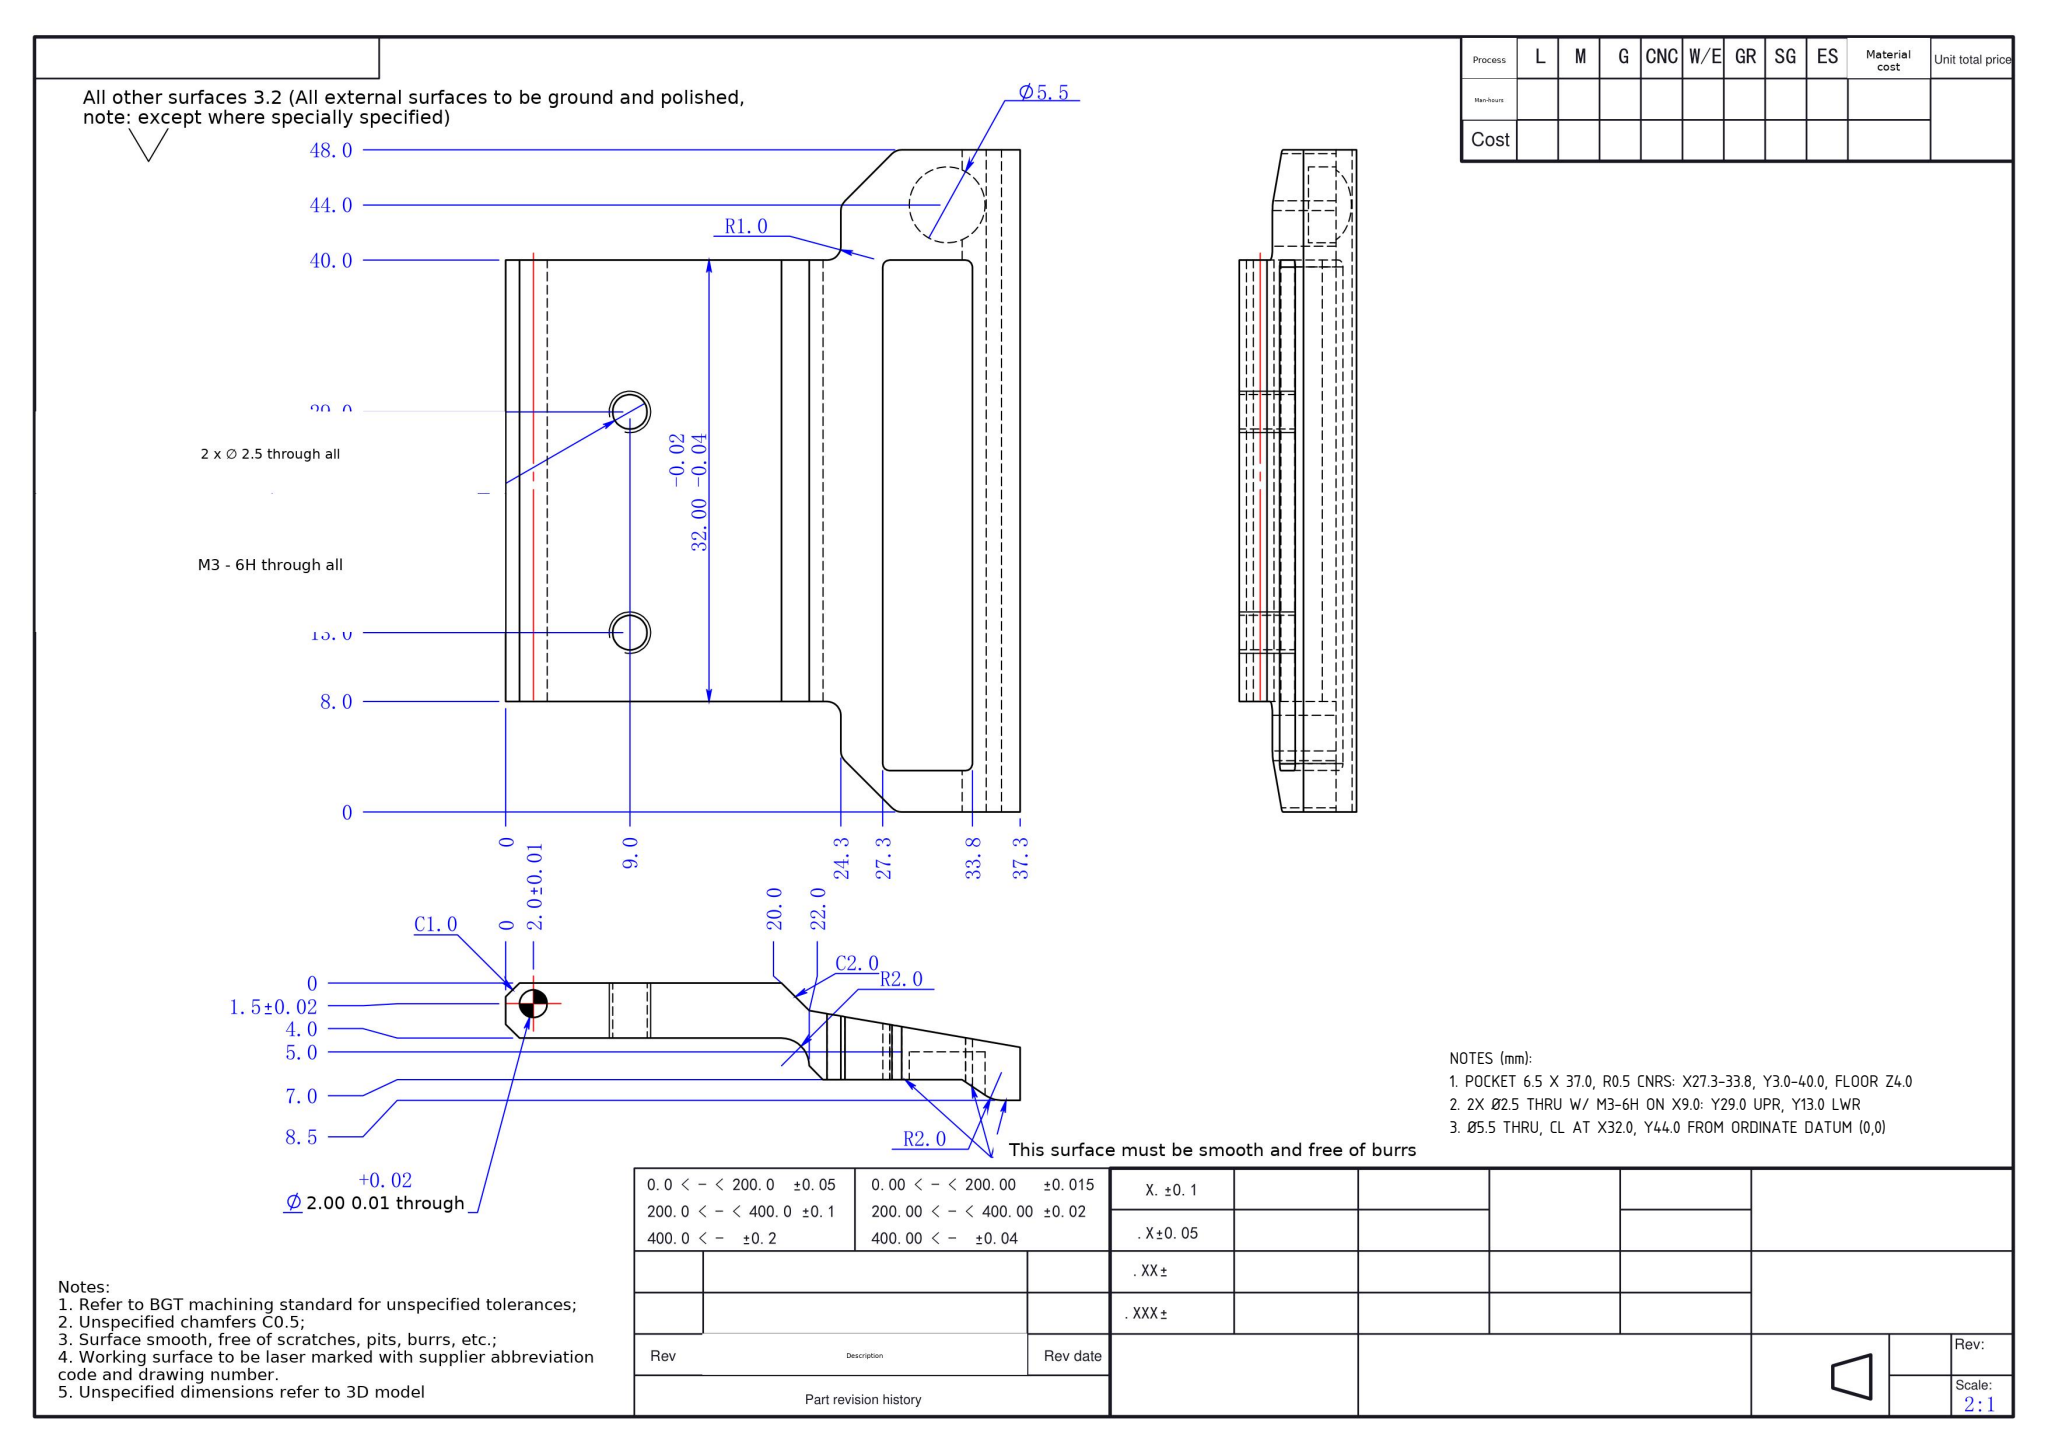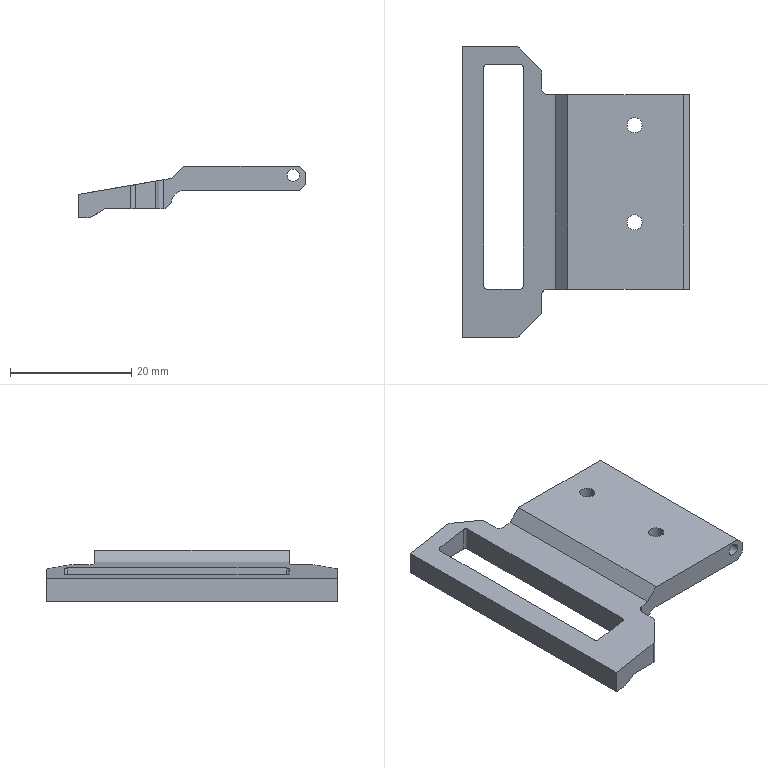Part | SolidWorks | mm | 1 solid | 45 faces | box 37.3 x 48 x 8.5 mm | volume 4364 mm3 | plane 25 | cylinder 20 | commonest cylinder face diameters 2 x8 2.5 x4 1 x4 5.5 x2 4 x2
Drawing notes:
POCKET 6.5 X 37.0, R0.5 CNRS: X27.3-33.8, Y3.0-40.0, FLOOR Z4.0 | from the solid: Ø1.0 (R0.5) cnr cyls at (3.96,8.5),(3.96,44.5),(9.46,8.5),(9.46,44.5); x-planes 3.46/9.96 -> X33.8/27.3; y-planes 8.0/45.0 -> Y40.0/3.0; z-plane 4.5 -> floor Z4.0
2X Ø2.5 THRU W/ M3-6H ON X9.0: Y29.0 UPR, Y13.0 LWR | from the solid: Ø2.5 THRU cyls, axis Z at (28.3,19.0) & (28.3,35.0); X=37.3-28.3=9.0, Y=48-19=29.0, Y=48-35=13.0
Ø5.5 THRU, CL AT X32.0, Y44.0 FROM ORDINATE DATUM (0,0) | from the solid: Ø5.5 cyl, axis Z at bbox (5.3,4.0); drawing datum flip: X=37.3-5.3=32.0, Y=48.0-4.0=44.0